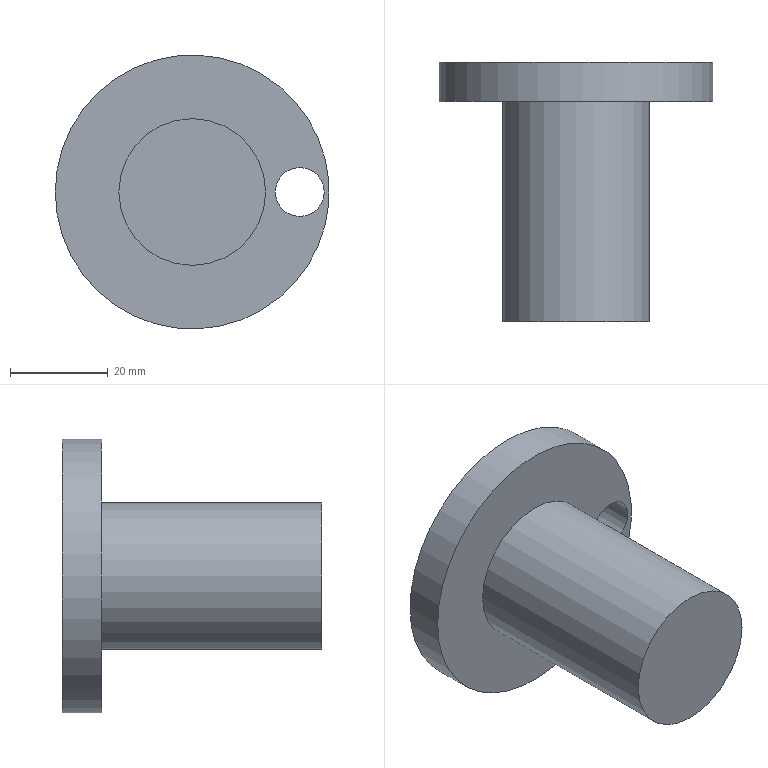Component | NX | MID_CYL_LOC_PIN | 1 solid | 6 faces | box 56 x 53 x 56 mm | volume 50884 mm3 | cylinder 3 | plane 3 | commonest cylinder face diameters 30 x1 56 x1 10 x1
STEP:
#1=CARTESIAN_POINT('',(0.,0.,0.));
#2=DIRECTION('',(0.,0.,1.));
#3=DIRECTION('',(1.,0.,0.));
#4=AXIS2_PLACEMENT_3D('',#1,#2,#3);
#5=CARTESIAN_POINT('',(-43.675,100.796,62.5));
#6=VERTEX_POINT('',#5);
#7=CARTESIAN_POINT('',(-28.675,100.796,62.5));
#8=DIRECTION('',(0.,1.,0.));
#9=DIRECTION('',(-1.,0.,0.));
#10=AXIS2_PLACEMENT_3D('',#7,#8,#9);
#11=CIRCLE('',#10,15.);
#12=CARTESIAN_POINT('',(-28.675,100.796,62.5));
#13=DIRECTION('',(0.,-1.,0.));
#14=DIRECTION('',(1.,0.,0.));
#15=AXIS2_PLACEMENT_3D('',#12,#13,#14);
#16=CYLINDRICAL_SURFACE('',#15,15.);
#17=CARTESIAN_POINT('',(9.425,0.));
#18=DIRECTION('',(-1.,0.));
#19=VECTOR('',#18,1.);
#20=LINE('',#17,#19);
#21=(GEOMETRIC_REPRESENTATION_CONTEXT(2)PARAMETRIC_REPRESENTATION_CONTEXT()REPRESENTATION_CONTEXT('',''));
#22=DEFINITIONAL_REPRESENTATION('',(#20),#21);
#23=PCURVE('',#16,#22);
#24=CARTESIAN_POINT('',(-28.675,100.796,62.5));
#25=DIRECTION('',(0.,-1.,0.));
#26=DIRECTION('',(1.,0.,0.));
#27=AXIS2_PLACEMENT_3D('',#24,#25,#26);
#28=PLANE('',#27);
#29=CARTESIAN_POINT('',(-15.,0.));
#30=CARTESIAN_POINT('',(-15.,25.981));
#31=CARTESIAN_POINT('',(7.5,12.99));
#32=CARTESIAN_POINT('',(30.,0.));
#33=CARTESIAN_POINT('',(7.5,-12.99));
#34=CARTESIAN_POINT('',(-15.,-25.981));
#35=CARTESIAN_POINT('',(-15.,0.));
#36=(BOUNDED_CURVE()B_SPLINE_CURVE(2,(#29,#30,#31,#32,#33,#34,#35),.UNSPECIFIED.,.T.,.F.)B_SPLINE_CURVE_WITH_KNOTS((1,2,2,2,2,1),(-2.094,0.,2.094,4.189,6.283,8.378),.UNSPECIFIED.)CURVE()GEOMETRIC_REPRESENTATION_ITEM()RATIONAL_B_SPLINE_CURVE((1.,0.5,1.,0.5,1.,0.5,1.))REPRESENTATION_ITEM(''));
#37=(GEOMETRIC_REPRESENTATION_CONTEXT(2)PARAMETRIC_REPRESENTATION_CONTEXT()REPRESENTATION_CONTEXT('',''));
#38=DEFINITIONAL_REPRESENTATION('',(#36),#37);
#39=PCURVE('',#28,#38);
#40=SURFACE_CURVE('',#11,(#23,#39),.PCURVE_S1.);
#41=EDGE_CURVE('',#6,#6,#40,.T.);
#42=ORIENTED_EDGE('',*,*,#41,.F.);
#43=CARTESIAN_POINT('',(-43.675,55.796,62.5));
#44=VERTEX_POINT('',#43);
#45=CARTESIAN_POINT('',(-43.675,100.796,62.5));
#46=CARTESIAN_POINT('',(-43.675,55.796,62.5));
#47=B_SPLINE_CURVE_WITH_KNOTS('',1,(#45,#46),.UNSPECIFIED.,.F.,.F.,(2,2),(0.,45.),.PIECEWISE_BEZIER_KNOTS.);
#48=CARTESIAN_POINT('',(9.425,0.));
#49=DIRECTION('',(0.,1.));
#50=VECTOR('',#49,1.);
#51=LINE('',#48,#50);
#52=(GEOMETRIC_REPRESENTATION_CONTEXT(2)PARAMETRIC_REPRESENTATION_CONTEXT()REPRESENTATION_CONTEXT('',''));
#53=DEFINITIONAL_REPRESENTATION('',(#51),#52);
#54=PCURVE('',#16,#53);
#55=CARTESIAN_POINT('',(3.142,0.));
#56=DIRECTION('',(0.,1.));
#57=VECTOR('',#56,1.);
#58=LINE('',#55,#57);
#59=(GEOMETRIC_REPRESENTATION_CONTEXT(2)PARAMETRIC_REPRESENTATION_CONTEXT()REPRESENTATION_CONTEXT('',''));
#60=DEFINITIONAL_REPRESENTATION('',(#58),#59);
#61=PCURVE('',#16,#60);
#62=SEAM_CURVE('',#47,(#54,#61),.PCURVE_S1.);
#63=EDGE_CURVE('',#6,#44,#62,.T.);
#64=ORIENTED_EDGE('',*,*,#63,.T.);
#65=CARTESIAN_POINT('',(-28.675,55.796,62.5));
#66=DIRECTION('',(0.,1.,0.));
#67=DIRECTION('',(-1.,0.,0.));
#68=AXIS2_PLACEMENT_3D('',#65,#66,#67);
#69=CIRCLE('',#68,15.);
#70=CARTESIAN_POINT('',(9.425,45.));
#71=DIRECTION('',(-1.,0.));
#72=VECTOR('',#71,1.);
#73=LINE('',#70,#72);
#74=(GEOMETRIC_REPRESENTATION_CONTEXT(2)PARAMETRIC_REPRESENTATION_CONTEXT()REPRESENTATION_CONTEXT('',''));
#75=DEFINITIONAL_REPRESENTATION('',(#73),#74);
#76=PCURVE('',#16,#75);
#77=CARTESIAN_POINT('',(-28.675,55.796,62.5));
#78=DIRECTION('',(0.,1.,0.));
#79=DIRECTION('',(-1.,0.,0.));
#80=AXIS2_PLACEMENT_3D('',#77,#78,#79);
#81=PLANE('',#80);
#82=CARTESIAN_POINT('',(0.,0.));
#83=DIRECTION('',(1.,0.));
#84=AXIS2_PLACEMENT_2D('',#82,#83);
#85=CIRCLE('',#84,15.);
#86=(GEOMETRIC_REPRESENTATION_CONTEXT(2)PARAMETRIC_REPRESENTATION_CONTEXT()REPRESENTATION_CONTEXT('',''));
#87=DEFINITIONAL_REPRESENTATION('',(#85),#86);
#88=PCURVE('',#81,#87);
#89=SURFACE_CURVE('',#69,(#76,#88),.PCURVE_S1.);
#90=EDGE_CURVE('',#44,#44,#89,.T.);
#91=ORIENTED_EDGE('',*,*,#90,.T.);
#92=ORIENTED_EDGE('',*,*,#63,.F.);
#93=EDGE_LOOP('',(#42,#64,#91,#92));
#94=FACE_BOUND('',#93,.T.);
#95=ADVANCED_FACE('',(#94),#16,.T.);
#96=ORIENTED_EDGE('',*,*,#90,.F.);
#97=EDGE_LOOP('',(#96));
#98=FACE_BOUND('',#97,.T.);
#99=ADVANCED_FACE('',(#98),#81,.F.);
#100=CARTESIAN_POINT('',(-56.675,108.796,62.5));
#101=VERTEX_POINT('',#100);
#102=CARTESIAN_POINT('',(-28.675,108.796,62.5));
#103=DIRECTION('',(0.,-1.,0.));
#104=DIRECTION('',(-1.,0.,0.));
#105=AXIS2_PLACEMENT_3D('',#102,#103,#104);
#106=CIRCLE('',#105,28.);
#107=CARTESIAN_POINT('',(-28.675,108.796,62.5));
#108=DIRECTION('',(0.,-1.,0.));
#109=DIRECTION('',(1.,0.,0.));
#110=AXIS2_PLACEMENT_3D('',#107,#108,#109);
#111=CYLINDRICAL_SURFACE('',#110,28.);
#112=CARTESIAN_POINT('',(3.142,0.));
#113=DIRECTION('',(1.,0.));
#114=VECTOR('',#113,1.);
#115=LINE('',#112,#114);
#116=(GEOMETRIC_REPRESENTATION_CONTEXT(2)PARAMETRIC_REPRESENTATION_CONTEXT()REPRESENTATION_CONTEXT('',''));
#117=DEFINITIONAL_REPRESENTATION('',(#115),#116);
#118=PCURVE('',#111,#117);
#119=CARTESIAN_POINT('',(-28.675,108.796,62.5));
#120=DIRECTION('',(0.,-1.,0.));
#121=DIRECTION('',(1.,0.,0.));
#122=AXIS2_PLACEMENT_3D('',#119,#120,#121);
#123=PLANE('',#122);
#124=CARTESIAN_POINT('',(0.,0.));
#125=DIRECTION('',(-1.,0.));
#126=AXIS2_PLACEMENT_2D('',#124,#125);
#127=CIRCLE('',#126,28.);
#128=(GEOMETRIC_REPRESENTATION_CONTEXT(2)PARAMETRIC_REPRESENTATION_CONTEXT()REPRESENTATION_CONTEXT('',''));
#129=DEFINITIONAL_REPRESENTATION('',(#127),#128);
#130=PCURVE('',#123,#129);
#131=SURFACE_CURVE('',#106,(#118,#130),.PCURVE_S1.);
#132=EDGE_CURVE('',#101,#101,#131,.T.);
#133=ORIENTED_EDGE('',*,*,#132,.T.);
#134=CARTESIAN_POINT('',(-56.675,100.796,62.5));
#135=VERTEX_POINT('',#134);
#136=CARTESIAN_POINT('',(-56.675,108.796,62.5));
#137=CARTESIAN_POINT('',(-56.675,100.796,62.5));
#138=B_SPLINE_CURVE_WITH_KNOTS('',1,(#136,#137),.UNSPECIFIED.,.F.,.F.,(2,2),(0.,8.),.PIECEWISE_BEZIER_KNOTS.);
#139=CARTESIAN_POINT('',(9.425,0.));
#140=DIRECTION('',(0.,1.));
#141=VECTOR('',#140,1.);
#142=LINE('',#139,#141);
#143=(GEOMETRIC_REPRESENTATION_CONTEXT(2)PARAMETRIC_REPRESENTATION_CONTEXT()REPRESENTATION_CONTEXT('',''));
#144=DEFINITIONAL_REPRESENTATION('',(#142),#143);
#145=PCURVE('',#111,#144);
#146=CARTESIAN_POINT('',(3.142,0.));
#147=DIRECTION('',(0.,1.));
#148=VECTOR('',#147,1.);
#149=LINE('',#146,#148);
#150=(GEOMETRIC_REPRESENTATION_CONTEXT(2)PARAMETRIC_REPRESENTATION_CONTEXT()REPRESENTATION_CONTEXT('',''));
#151=DEFINITIONAL_REPRESENTATION('',(#149),#150);
#152=PCURVE('',#111,#151);
#153=SEAM_CURVE('',#138,(#145,#152),.PCURVE_S1.);
#154=EDGE_CURVE('',#101,#135,#153,.T.);
#155=ORIENTED_EDGE('',*,*,#154,.T.);
#156=CARTESIAN_POINT('',(-28.675,100.796,62.5));
#157=DIRECTION('',(0.,-1.,0.));
#158=DIRECTION('',(-1.,0.,0.));
#159=AXIS2_PLACEMENT_3D('',#156,#157,#158);
#160=CIRCLE('',#159,28.);
#161=CARTESIAN_POINT('',(3.142,8.));
#162=DIRECTION('',(1.,0.));
#163=VECTOR('',#162,1.);
#164=LINE('',#161,#163);
#165=(GEOMETRIC_REPRESENTATION_CONTEXT(2)PARAMETRIC_REPRESENTATION_CONTEXT()REPRESENTATION_CONTEXT('',''));
#166=DEFINITIONAL_REPRESENTATION('',(#164),#165);
#167=PCURVE('',#111,#166);
#168=CARTESIAN_POINT('',(0.,0.));
#169=DIRECTION('',(-1.,0.));
#170=AXIS2_PLACEMENT_2D('',#168,#169);
#171=CIRCLE('',#170,28.);
#172=(GEOMETRIC_REPRESENTATION_CONTEXT(2)PARAMETRIC_REPRESENTATION_CONTEXT()REPRESENTATION_CONTEXT('',''));
#173=DEFINITIONAL_REPRESENTATION('',(#171),#172);
#174=PCURVE('',#28,#173);
#175=SURFACE_CURVE('',#160,(#167,#174),.PCURVE_S1.);
#176=EDGE_CURVE('',#135,#135,#175,.T.);
#177=ORIENTED_EDGE('',*,*,#176,.F.);
#178=ORIENTED_EDGE('',*,*,#154,.F.);
#179=EDGE_LOOP('',(#133,#155,#177,#178));
#180=FACE_BOUND('',#179,.T.);
#181=ADVANCED_FACE('',(#180),#111,.T.);
#182=CARTESIAN_POINT('',(-11.675,108.796,62.5));
#183=VERTEX_POINT('',#182);
#184=CARTESIAN_POINT('',(-6.675,108.796,62.5));
#185=DIRECTION('',(0.,-1.,0.));
#186=DIRECTION('',(-1.,0.,0.));
#187=AXIS2_PLACEMENT_3D('',#184,#185,#186);
#188=CIRCLE('',#187,5.);
#189=CARTESIAN_POINT('',(22.,0.));
#190=DIRECTION('',(-1.,0.));
#191=AXIS2_PLACEMENT_2D('',#189,#190);
#192=CIRCLE('',#191,5.);
#193=(GEOMETRIC_REPRESENTATION_CONTEXT(2)PARAMETRIC_REPRESENTATION_CONTEXT()REPRESENTATION_CONTEXT('',''));
#194=DEFINITIONAL_REPRESENTATION('',(#192),#193);
#195=PCURVE('',#123,#194);
#196=CARTESIAN_POINT('',(-6.675,88.796,62.5));
#197=DIRECTION('',(0.,1.,0.));
#198=DIRECTION('',(-1.,0.,0.));
#199=AXIS2_PLACEMENT_3D('',#196,#197,#198);
#200=CYLINDRICAL_SURFACE('',#199,5.);
#201=CARTESIAN_POINT('',(6.283,20.));
#202=DIRECTION('',(-1.,0.));
#203=VECTOR('',#202,1.);
#204=LINE('',#201,#203);
#205=(GEOMETRIC_REPRESENTATION_CONTEXT(2)PARAMETRIC_REPRESENTATION_CONTEXT()REPRESENTATION_CONTEXT('',''));
#206=DEFINITIONAL_REPRESENTATION('',(#204),#205);
#207=PCURVE('',#200,#206);
#208=SURFACE_CURVE('',#188,(#195,#207),.PCURVE_S1.);
#209=EDGE_CURVE('',#183,#183,#208,.T.);
#210=ORIENTED_EDGE('',*,*,#209,.T.);
#211=EDGE_LOOP('',(#210));
#212=FACE_BOUND('',#211,.T.);
#213=ORIENTED_EDGE('',*,*,#132,.F.);
#214=EDGE_LOOP('',(#213));
#215=FACE_BOUND('',#214,.T.);
#216=ADVANCED_FACE('',(#212,#215),#123,.F.);
#217=CARTESIAN_POINT('',(-1.675,100.796,62.5));
#218=VERTEX_POINT('',#217);
#219=CARTESIAN_POINT('',(-11.675,100.796,62.5));
#220=VERTEX_POINT('',#219);
#221=CARTESIAN_POINT('',(-6.675,100.796,62.5));
#222=DIRECTION('',(0.,1.,0.));
#223=DIRECTION('',(1.,0.,0.));
#224=AXIS2_PLACEMENT_3D('',#221,#222,#223);
#225=CIRCLE('',#224,5.);
#226=CARTESIAN_POINT('',(27.,0.));
#227=CARTESIAN_POINT('',(27.,-8.66));
#228=CARTESIAN_POINT('',(19.5,-4.33));
#229=CARTESIAN_POINT('',(12.,-0.));
#230=CARTESIAN_POINT('',(19.5,4.33));
#231=CARTESIAN_POINT('',(27.,8.66));
#232=CARTESIAN_POINT('',(27.,0.));
#233=(BOUNDED_CURVE()B_SPLINE_CURVE(2,(#226,#227,#228,#229,#230,#231,#232),.UNSPECIFIED.,.T.,.F.)B_SPLINE_CURVE_WITH_KNOTS((1,2,2,2,2,1),(-2.094,0.,2.094,4.189,6.283,8.378),.UNSPECIFIED.)CURVE()GEOMETRIC_REPRESENTATION_ITEM()RATIONAL_B_SPLINE_CURVE((1.,0.5,1.,0.5,1.,0.5,1.))REPRESENTATION_ITEM(''));
#234=(GEOMETRIC_REPRESENTATION_CONTEXT(2)PARAMETRIC_REPRESENTATION_CONTEXT()REPRESENTATION_CONTEXT('',''));
#235=DEFINITIONAL_REPRESENTATION('',(#233),#234);
#236=PCURVE('',#28,#235);
#237=CARTESIAN_POINT('',(3.142,12.));
#238=DIRECTION('',(1.,0.));
#239=VECTOR('',#238,1.);
#240=LINE('',#237,#239);
#241=(GEOMETRIC_REPRESENTATION_CONTEXT(2)PARAMETRIC_REPRESENTATION_CONTEXT()REPRESENTATION_CONTEXT('',''));
#242=DEFINITIONAL_REPRESENTATION('',(#240),#241);
#243=PCURVE('',#200,#242);
#244=SURFACE_CURVE('',#225,(#236,#243),.PCURVE_S1.);
#245=EDGE_CURVE('',#218,#220,#244,.T.);
#246=ORIENTED_EDGE('',*,*,#245,.T.);
#247=CARTESIAN_POINT('',(-6.675,100.796,62.5));
#248=DIRECTION('',(0.,1.,0.));
#249=DIRECTION('',(1.,0.,0.));
#250=AXIS2_PLACEMENT_3D('',#247,#248,#249);
#251=CIRCLE('',#250,5.);
#252=CARTESIAN_POINT('',(27.,0.));
#253=CARTESIAN_POINT('',(27.,-8.66));
#254=CARTESIAN_POINT('',(19.5,-4.33));
#255=CARTESIAN_POINT('',(12.,-0.));
#256=CARTESIAN_POINT('',(19.5,4.33));
#257=CARTESIAN_POINT('',(27.,8.66));
#258=CARTESIAN_POINT('',(27.,0.));
#259=(BOUNDED_CURVE()B_SPLINE_CURVE(2,(#252,#253,#254,#255,#256,#257,#258),.UNSPECIFIED.,.T.,.F.)B_SPLINE_CURVE_WITH_KNOTS((1,2,2,2,2,1),(-2.094,0.,2.094,4.189,6.283,8.378),.UNSPECIFIED.)CURVE()GEOMETRIC_REPRESENTATION_ITEM()RATIONAL_B_SPLINE_CURVE((1.,0.5,1.,0.5,1.,0.5,1.))REPRESENTATION_ITEM(''));
#260=(GEOMETRIC_REPRESENTATION_CONTEXT(2)PARAMETRIC_REPRESENTATION_CONTEXT()REPRESENTATION_CONTEXT('',''));
#261=DEFINITIONAL_REPRESENTATION('',(#259),#260);
#262=PCURVE('',#28,#261);
#263=CARTESIAN_POINT('',(-3.142,12.));
#264=DIRECTION('',(1.,0.));
#265=VECTOR('',#264,1.);
#266=LINE('',#263,#265);
#267=(GEOMETRIC_REPRESENTATION_CONTEXT(2)PARAMETRIC_REPRESENTATION_CONTEXT()REPRESENTATION_CONTEXT('',''));
#268=DEFINITIONAL_REPRESENTATION('',(#266),#267);
#269=PCURVE('',#200,#268);
#270=SURFACE_CURVE('',#251,(#262,#269),.PCURVE_S1.);
#271=EDGE_CURVE('',#220,#218,#270,.T.);
#272=ORIENTED_EDGE('',*,*,#271,.T.);
#273=EDGE_LOOP('',(#246,#272));
#274=FACE_BOUND('',#273,.T.);
#275=ORIENTED_EDGE('',*,*,#41,.T.);
#276=EDGE_LOOP('',(#275));
#277=FACE_BOUND('',#276,.T.);
#278=ORIENTED_EDGE('',*,*,#176,.T.);
#279=EDGE_LOOP('',(#278));
#280=FACE_BOUND('',#279,.T.);
#281=ADVANCED_FACE('',(#274,#277,#280),#28,.T.);
#282=ORIENTED_EDGE('',*,*,#245,.T.);
#283=CARTESIAN_POINT('',(-11.675,100.796,62.5));
#284=CARTESIAN_POINT('',(-11.675,108.796,62.5));
#285=B_SPLINE_CURVE_WITH_KNOTS('',1,(#283,#284),.UNSPECIFIED.,.F.,.F.,(2,2),(12.,20.),.PIECEWISE_BEZIER_KNOTS.);
#286=CARTESIAN_POINT('',(6.283,0.));
#287=DIRECTION('',(0.,1.));
#288=VECTOR('',#287,1.);
#289=LINE('',#286,#288);
#290=(GEOMETRIC_REPRESENTATION_CONTEXT(2)PARAMETRIC_REPRESENTATION_CONTEXT()REPRESENTATION_CONTEXT('',''));
#291=DEFINITIONAL_REPRESENTATION('',(#289),#290);
#292=PCURVE('',#200,#291);
#293=CARTESIAN_POINT('',(0.,0.));
#294=DIRECTION('',(0.,1.));
#295=VECTOR('',#294,1.);
#296=LINE('',#293,#295);
#297=(GEOMETRIC_REPRESENTATION_CONTEXT(2)PARAMETRIC_REPRESENTATION_CONTEXT()REPRESENTATION_CONTEXT('',''));
#298=DEFINITIONAL_REPRESENTATION('',(#296),#297);
#299=PCURVE('',#200,#298);
#300=SEAM_CURVE('',#285,(#292,#299),.PCURVE_S1.);
#301=EDGE_CURVE('',#220,#183,#300,.T.);
#302=ORIENTED_EDGE('',*,*,#301,.T.);
#303=ORIENTED_EDGE('',*,*,#209,.T.);
#304=ORIENTED_EDGE('',*,*,#301,.F.);
#305=ORIENTED_EDGE('',*,*,#271,.T.);
#306=EDGE_LOOP('',(#282,#302,#303,#304,#305));
#307=FACE_BOUND('',#306,.F.);
#308=ADVANCED_FACE('',(#307),#200,.F.);
#309=CLOSED_SHELL('',(#95,#99,#181,#216,#281,#308));
#310=MANIFOLD_SOLID_BREP('',#309);
#311=(LENGTH_UNIT()NAMED_UNIT(*)SI_UNIT(.MILLI.,.METRE.));
#312=UNCERTAINTY_MEASURE_WITH_UNIT(LENGTH_MEASURE(0.000005),#311,'','');
#313=(NAMED_UNIT(*)PLANE_ANGLE_UNIT()SI_UNIT($,.RADIAN.));
#314=(NAMED_UNIT(*)SI_UNIT($,.STERADIAN.)SOLID_ANGLE_UNIT());
#315=(GEOMETRIC_REPRESENTATION_CONTEXT(3)GLOBAL_UNCERTAINTY_ASSIGNED_CONTEXT((#312))GLOBAL_UNIT_ASSIGNED_CONTEXT((#311,#313,#314))REPRESENTATION_CONTEXT('',''));
#316=ADVANCED_BREP_SHAPE_REPRESENTATION('',(#4,#310),#315);